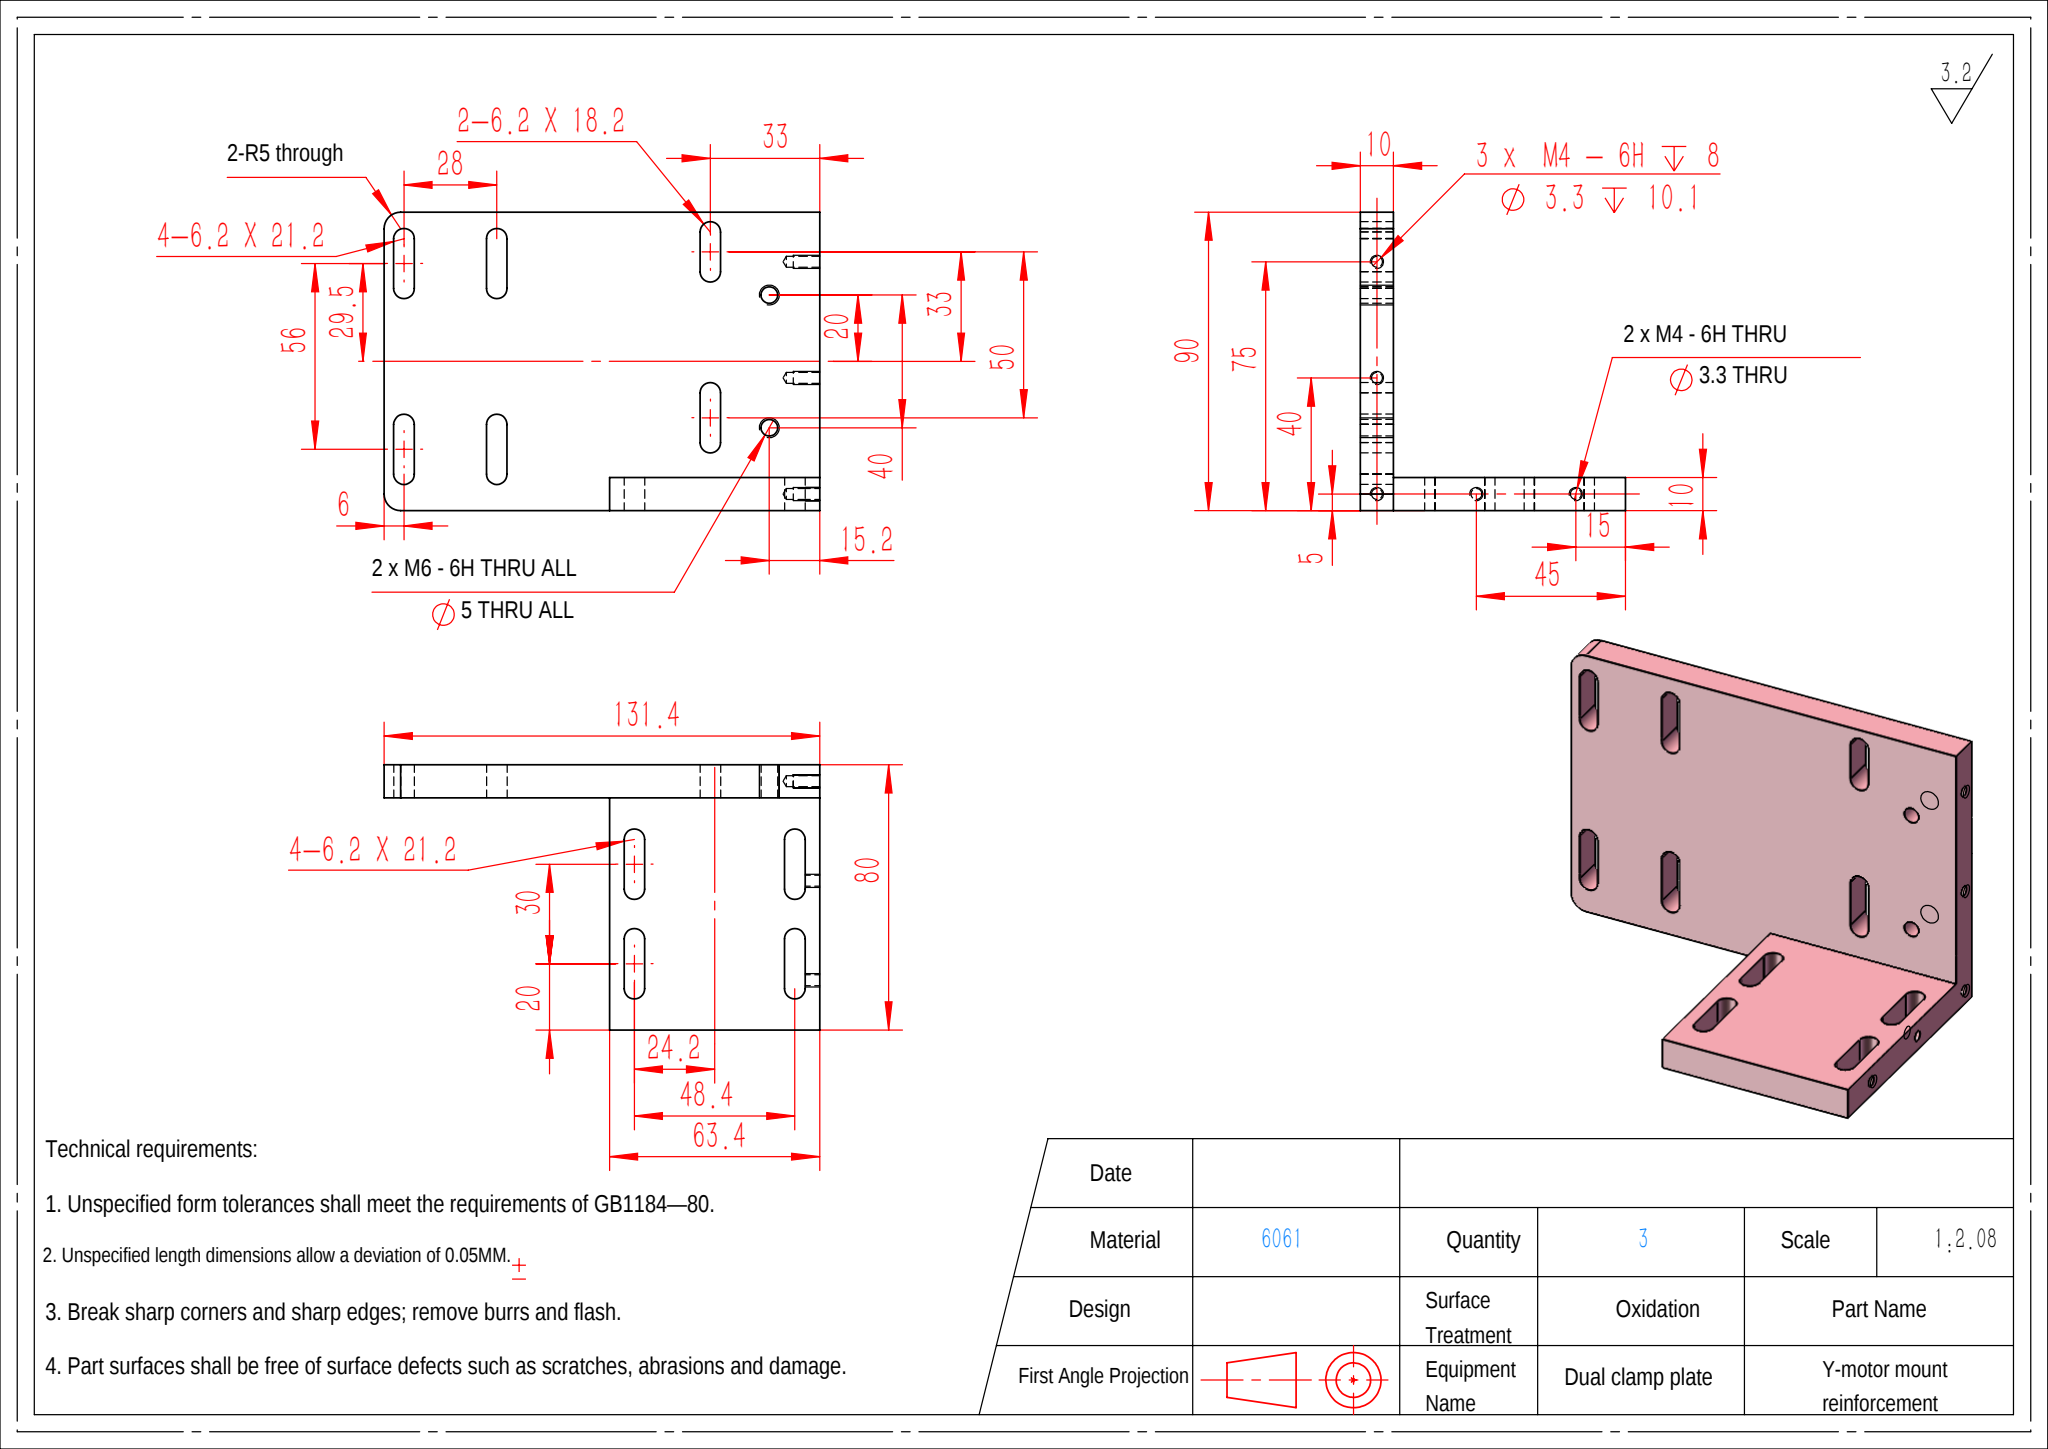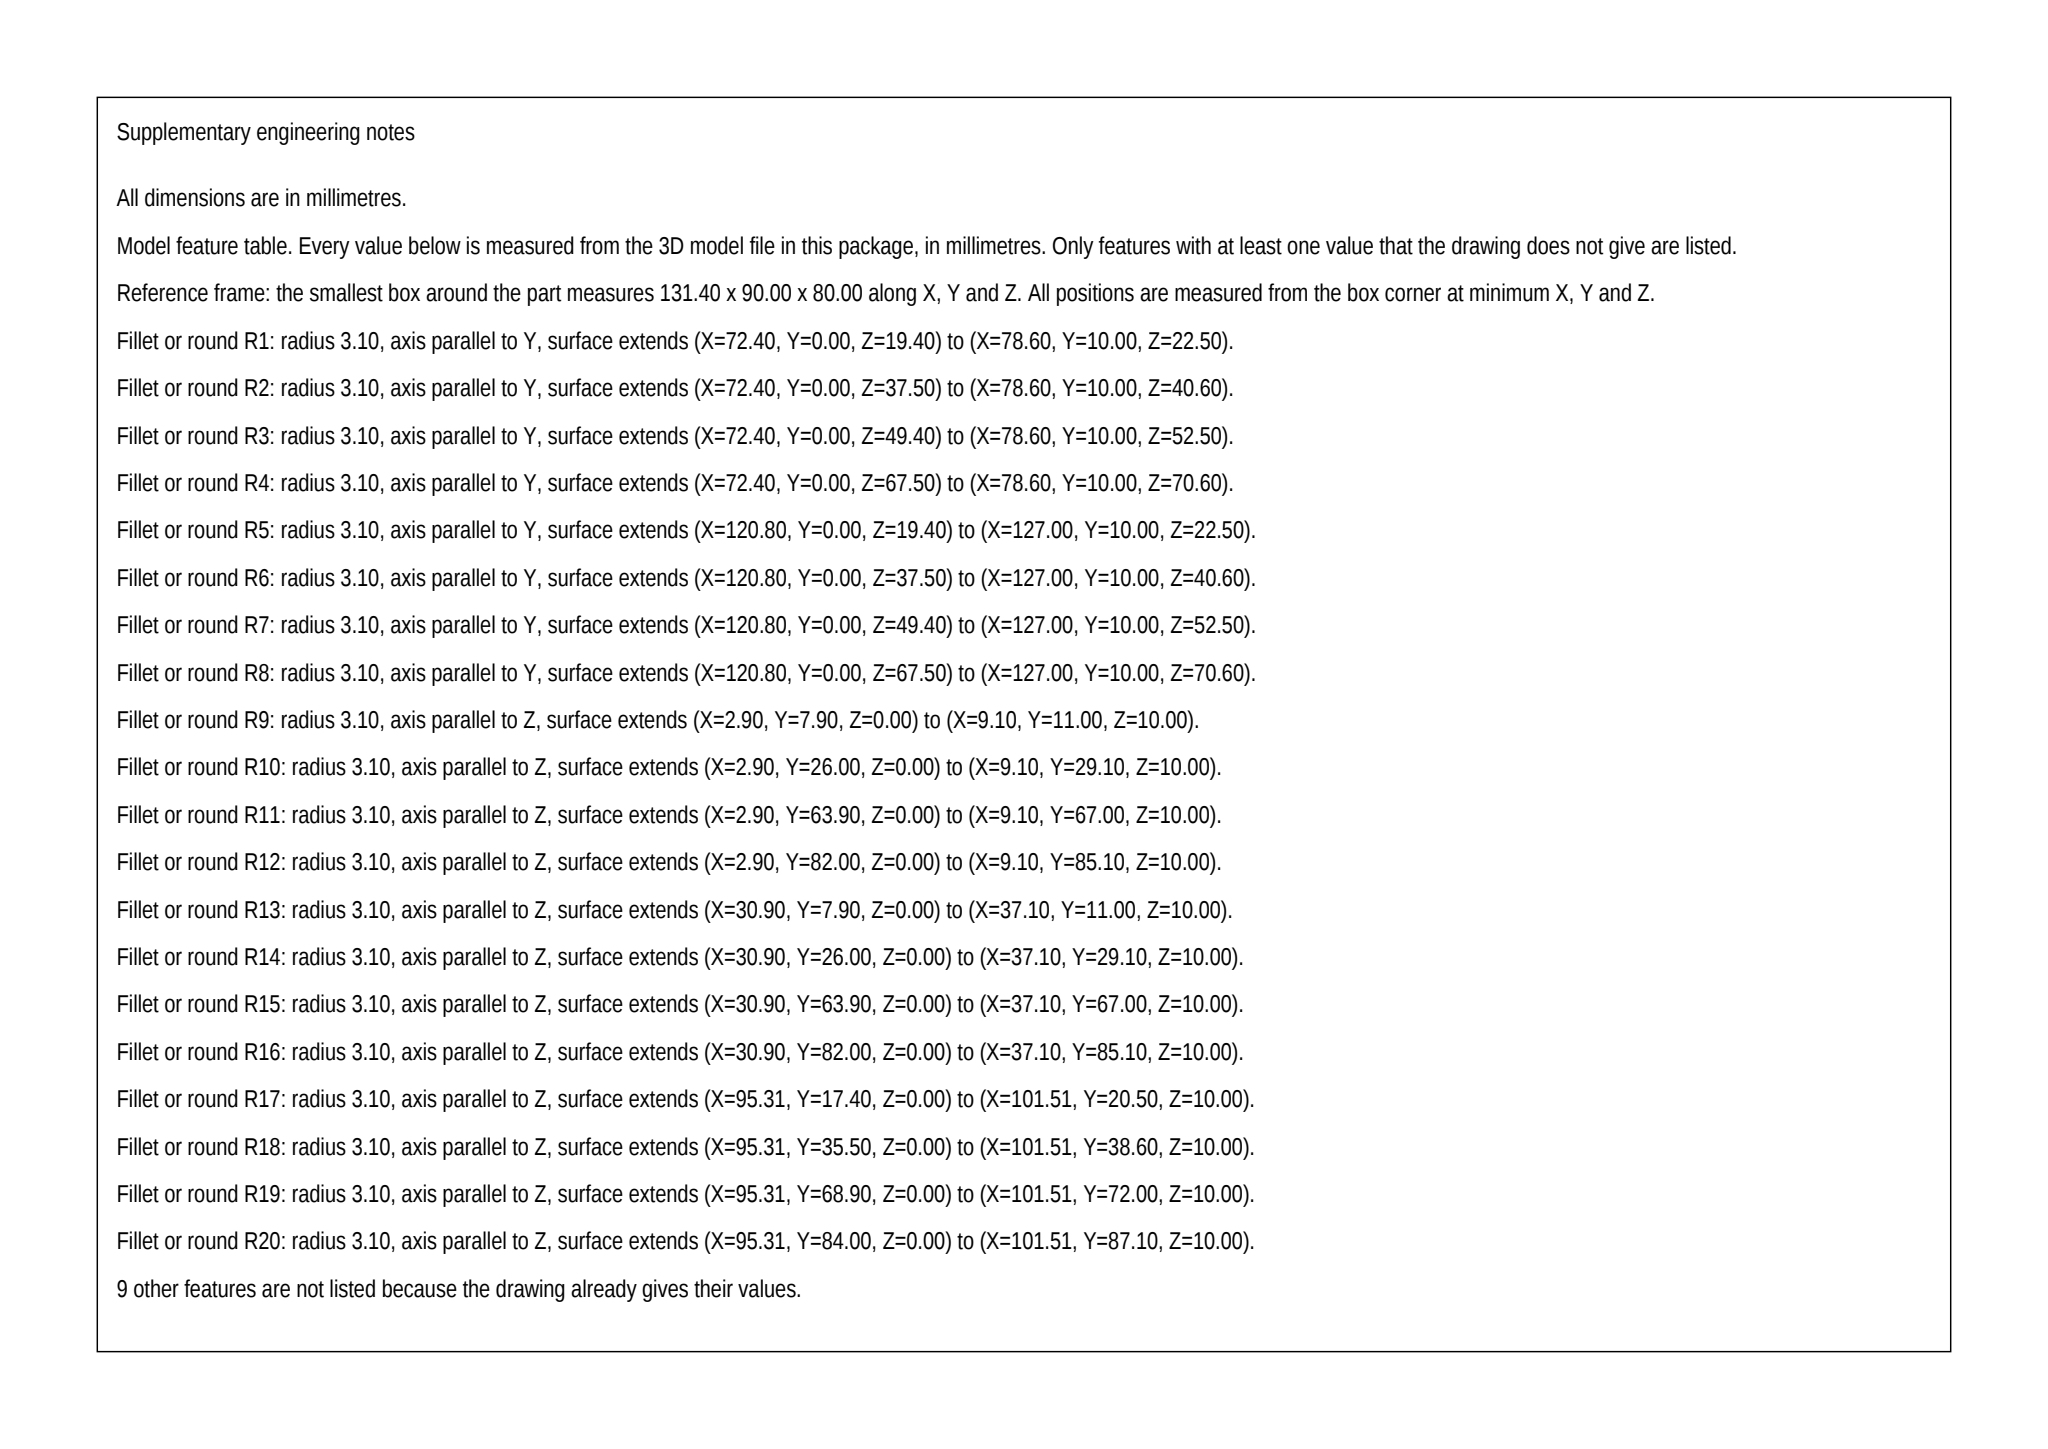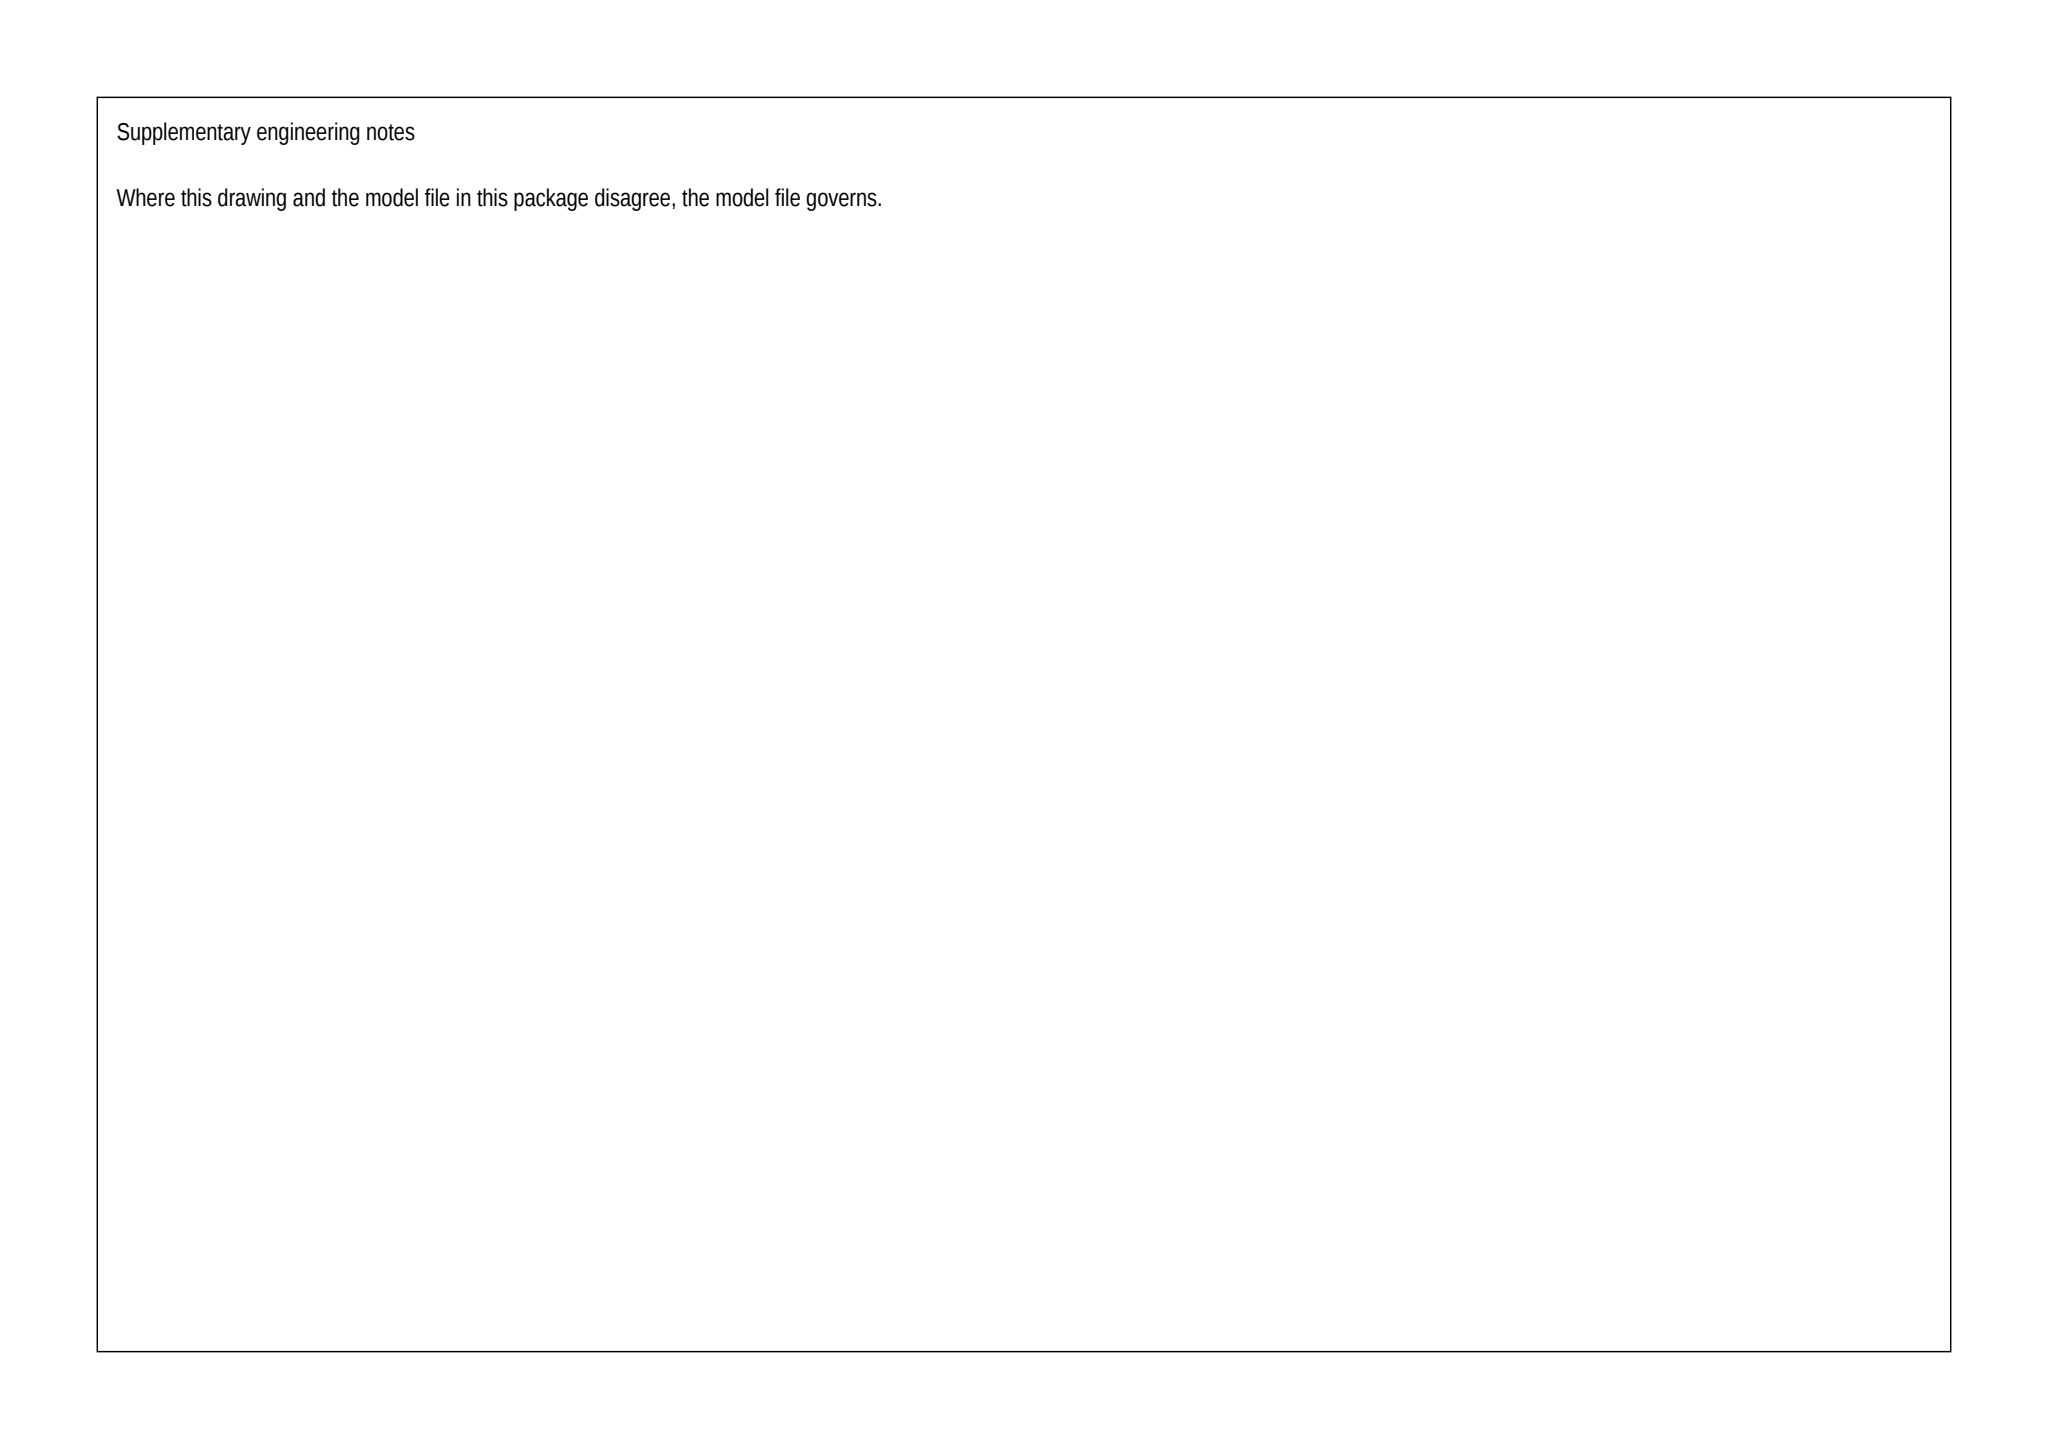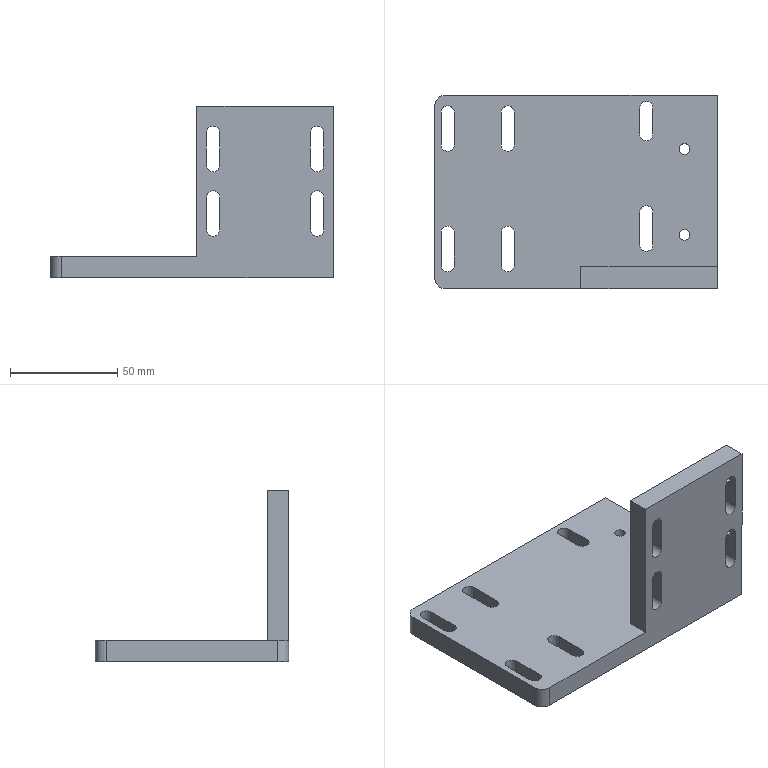Part | SolidWorks | mm | material 6061 | 1 solid | 75 faces | box 131.4 x 90 x 80 mm | volume 149664 mm3 | cylinder 40 | plane 29 | cone 6 | commonest cylinder face diameters 6.2 x24 3.3 x10 5 x4 10 x2
build123d program:
from build123d import *

# Parameters (mm, degrees)
SKETCH1_W                  = 131.4
SKETCH1_H                  = 90
BOSS_EXTRUDE1_DEPTH        = 10
CUT_EXTRUDE1_DEPTH         = 81.259
CUT_EXTRUDE2_DEPTH         = 81.259
CUT_EXTRUDE3_DEPTH         = 81.259
SKETCH7_W                  = 63.4
SKETCH7_H                  = 10
BOSS_EXTRUDE2_DEPTH        = 70
CUT_EXTRUDE7_DEPTH         = 131.83
SKETCH15_W                 = 1.65
SKETCH15_H                 = 4.4
M4_TAPPED_HOLE1_AT_2_COUNT = 2
M4_TAPPED_HOLE1_AT_2_PITCH = 30
M4_TAPPED_HOLE2_D          = 3.3
M4_TAPPED_HOLE2_DEPTH      = 10.1
M4_TAPPED_HOLE2_TIP        = 0.9914
M6_TAPPED_HOLE1_D          = 5
FILLET1_R                  = 5
LPATTERN2_COUNT            = 2
LPATTERN2_PITCH            = 28
LPATTERN2_COUNT_DIR2       = 2
LPATTERN2_PITCH_DIR2       = 56
LPATTERN3_COUNT            = 2
LPATTERN3_PITCH            = 30
LPATTERN3_COUNT_DIR2       = 2
LPATTERN3_PITCH_DIR2       = 48.4


with BuildPart() as part:
    # Sketch1 → Boss-Extrude1 (new body)
    with BuildSketch(Plane(origin=(0, 0, 0), x_dir=(-1, 0, 0), z_dir=(0, 0, -1))):
        Rectangle(SKETCH1_W, SKETCH1_H)
    extrude(amount=-BOSS_EXTRUDE1_DEPTH)

    # Sketch2 → Cut-Extrude1 (cut, through all)
    with BuildSketch(Plane(origin=(0, 0, 0), x_dir=(-1, 0, 0), z_dir=(0, 0, -1))):
        with BuildLine():
            Line((34.8, 37), (34.8, 22))
            ThreePointArc((34.8, 22), (31.7, 18.9), (28.6, 22))
            Line((28.6, 22), (28.6, 37))
            ThreePointArc((28.6, 37), (31.7, 40.1), (34.8, 37))
        make_face()
    cut_extrude1 = extrude(amount=-CUT_EXTRUDE1_DEPTH, mode=Mode.SUBTRACT)

    # Sketch3 → Cut-Extrude2 (cut, through all)
    with BuildSketch(Plane(origin=(0, 0, 0), x_dir=(-1, 0, 0), z_dir=(0, 0, -1))):
        with BuildLine():
            Line((-29.61, 39), (-29.61, 27))
            ThreePointArc((-29.61, 27), (-32.71, 23.9), (-35.81, 27))
            Line((-35.81, 27), (-35.81, 39))
            ThreePointArc((-35.81, 39), (-32.71, 42.1), (-29.61, 39))
        make_face()
    extrude(amount=-CUT_EXTRUDE2_DEPTH, mode=Mode.SUBTRACT)

    # Sketch4 → Cut-Extrude3 (cut, through all)
    with BuildSketch(Plane(origin=(0, 0, 0), x_dir=(-1, 0, 0), z_dir=(0, 0, -1))):
        with BuildLine():
            Line((-29.61, -9.5), (-29.61, -24.5))
            ThreePointArc((-29.61, -24.5), (-32.71, -27.6), (-35.81, -24.5))
            Line((-35.81, -24.5), (-35.81, -9.5))
            ThreePointArc((-35.81, -9.5), (-32.71, -6.4), (-29.61, -9.5))
        make_face()
    extrude(amount=-CUT_EXTRUDE3_DEPTH, mode=Mode.SUBTRACT)

    # Sketch7 → Boss-Extrude2 (add)
    with BuildSketch(Plane.XY.offset(10)):
        with Locations((34, -40)):
            Rectangle(SKETCH7_W, SKETCH7_H)
    extrude(amount=BOSS_EXTRUDE2_DEPTH)

    # Sketch9 → Cut-Extrude7 (cut, through all)
    with BuildSketch(Plane(origin=(0, -35, 0), x_dir=(-1, 0, 0), z_dir=(0, 1, 0))):
        with BuildLine():
            Line((-55.1, 37.5), (-55.1, 22.5))
            ThreePointArc((-55.1, 22.5), (-58.2, 19.4), (-61.3, 22.5))
            Line((-61.3, 22.5), (-61.3, 37.5))
            ThreePointArc((-61.3, 37.5), (-58.2, 40.6), (-55.1, 37.5))
        make_face()
    cut_extrude7 = extrude(amount=-CUT_EXTRUDE7_DEPTH, mode=Mode.SUBTRACT)

    # Sketch15 → M4 Tapped Hole1 (revolve, cut)
    with BuildSketch(Plane(origin=(61.3, -40, 35), x_dir=(0, 0, 1), z_dir=(0, 1, 0))):
        with Locations((0.825, 2.2)):
            Rectangle(SKETCH15_W, SKETCH15_H)
    m4_tapped_hole1 = revolve(axis=Axis((54.95, -40, 35), (1, 0, 0)), mode=Mode.SUBTRACT)

    # M4 Tapped Hole1 at 2: M4 Tapped Hole1 ×2
    with Locations(*[(0, 0, i * M4_TAPPED_HOLE1_AT_2_PITCH) for i in range(1, M4_TAPPED_HOLE1_AT_2_COUNT)]):
        add(m4_tapped_hole1, mode=Mode.SUBTRACT)

    # M4 Tapped Hole2
    with Locations(Plane(origin=(65.7, 0, 0), x_dir=(0, 0, -1), z_dir=(1, 0, 0))):
        with Locations((-5, 30), (-5, -5), (-5, -40)):
            Hole(M4_TAPPED_HOLE2_D / 2, depth=M4_TAPPED_HOLE2_DEPTH)
            with Locations((0, 0, -(M4_TAPPED_HOLE2_DEPTH + M4_TAPPED_HOLE2_TIP / 2))):  # 118° drill point
                Cone(0, M4_TAPPED_HOLE2_D / 2, M4_TAPPED_HOLE2_TIP, mode=Mode.SUBTRACT)

    # M6 Tapped Hole1 (through all)
    with Locations(Plane(origin=(0, 0, 0), x_dir=(-1, 0, 0), z_dir=(0, 0, -1))):
        with Locations((-50.5, 20), (-50.5, -20)):
            Hole(M6_TAPPED_HOLE1_D / 2)

    # Fillet1
    fillet1_edges = [part.edges().sort_by_distance(p)[0] for p in [
        (-65.7, 45, 5),
        (-65.7, -45, 5),
    ]]
    fillet(fillet1_edges, radius=FILLET1_R)

    # LPattern2: Cut-Extrude1 2 × 2
    with Locations(*[(-i * LPATTERN2_PITCH, -j * LPATTERN2_PITCH_DIR2, 0) for i in range(LPATTERN2_COUNT) for j in range(LPATTERN2_COUNT_DIR2) if (i, j) != (0, 0)]):
        add(cut_extrude1, mode=Mode.SUBTRACT)

    # LPattern3: Cut-Extrude7 2 × 2
    with Locations(*[(-j * LPATTERN3_PITCH_DIR2, 0, i * LPATTERN3_PITCH) for i in range(LPATTERN3_COUNT) for j in range(LPATTERN3_COUNT_DIR2) if (i, j) != (0, 0)]):
        add(cut_extrude7, mode=Mode.SUBTRACT)


solid = part.part